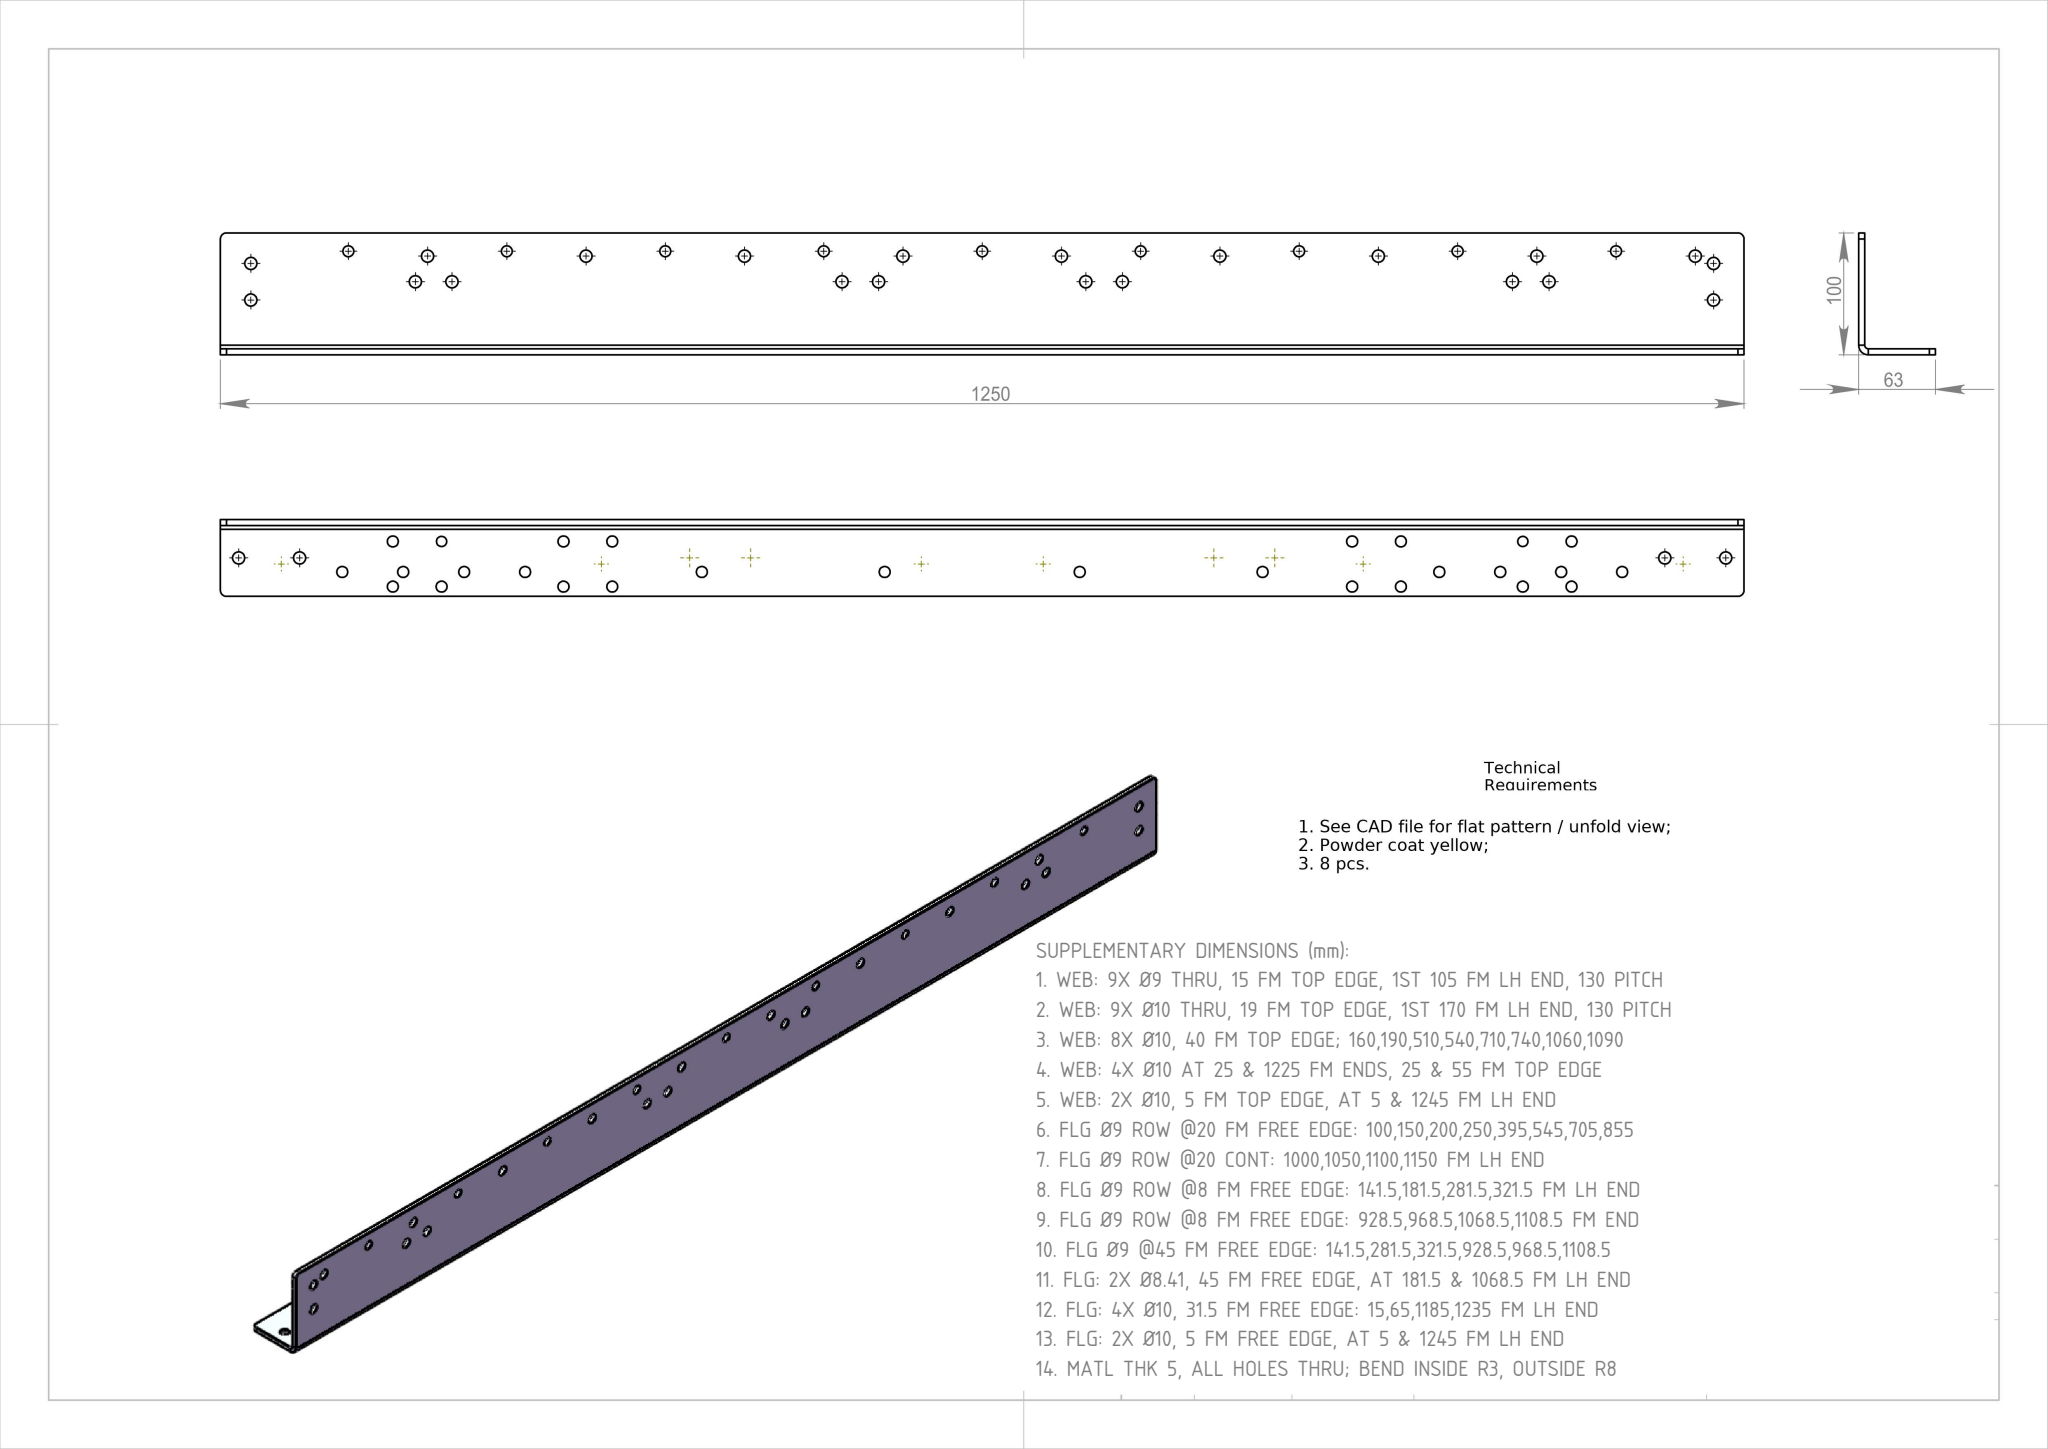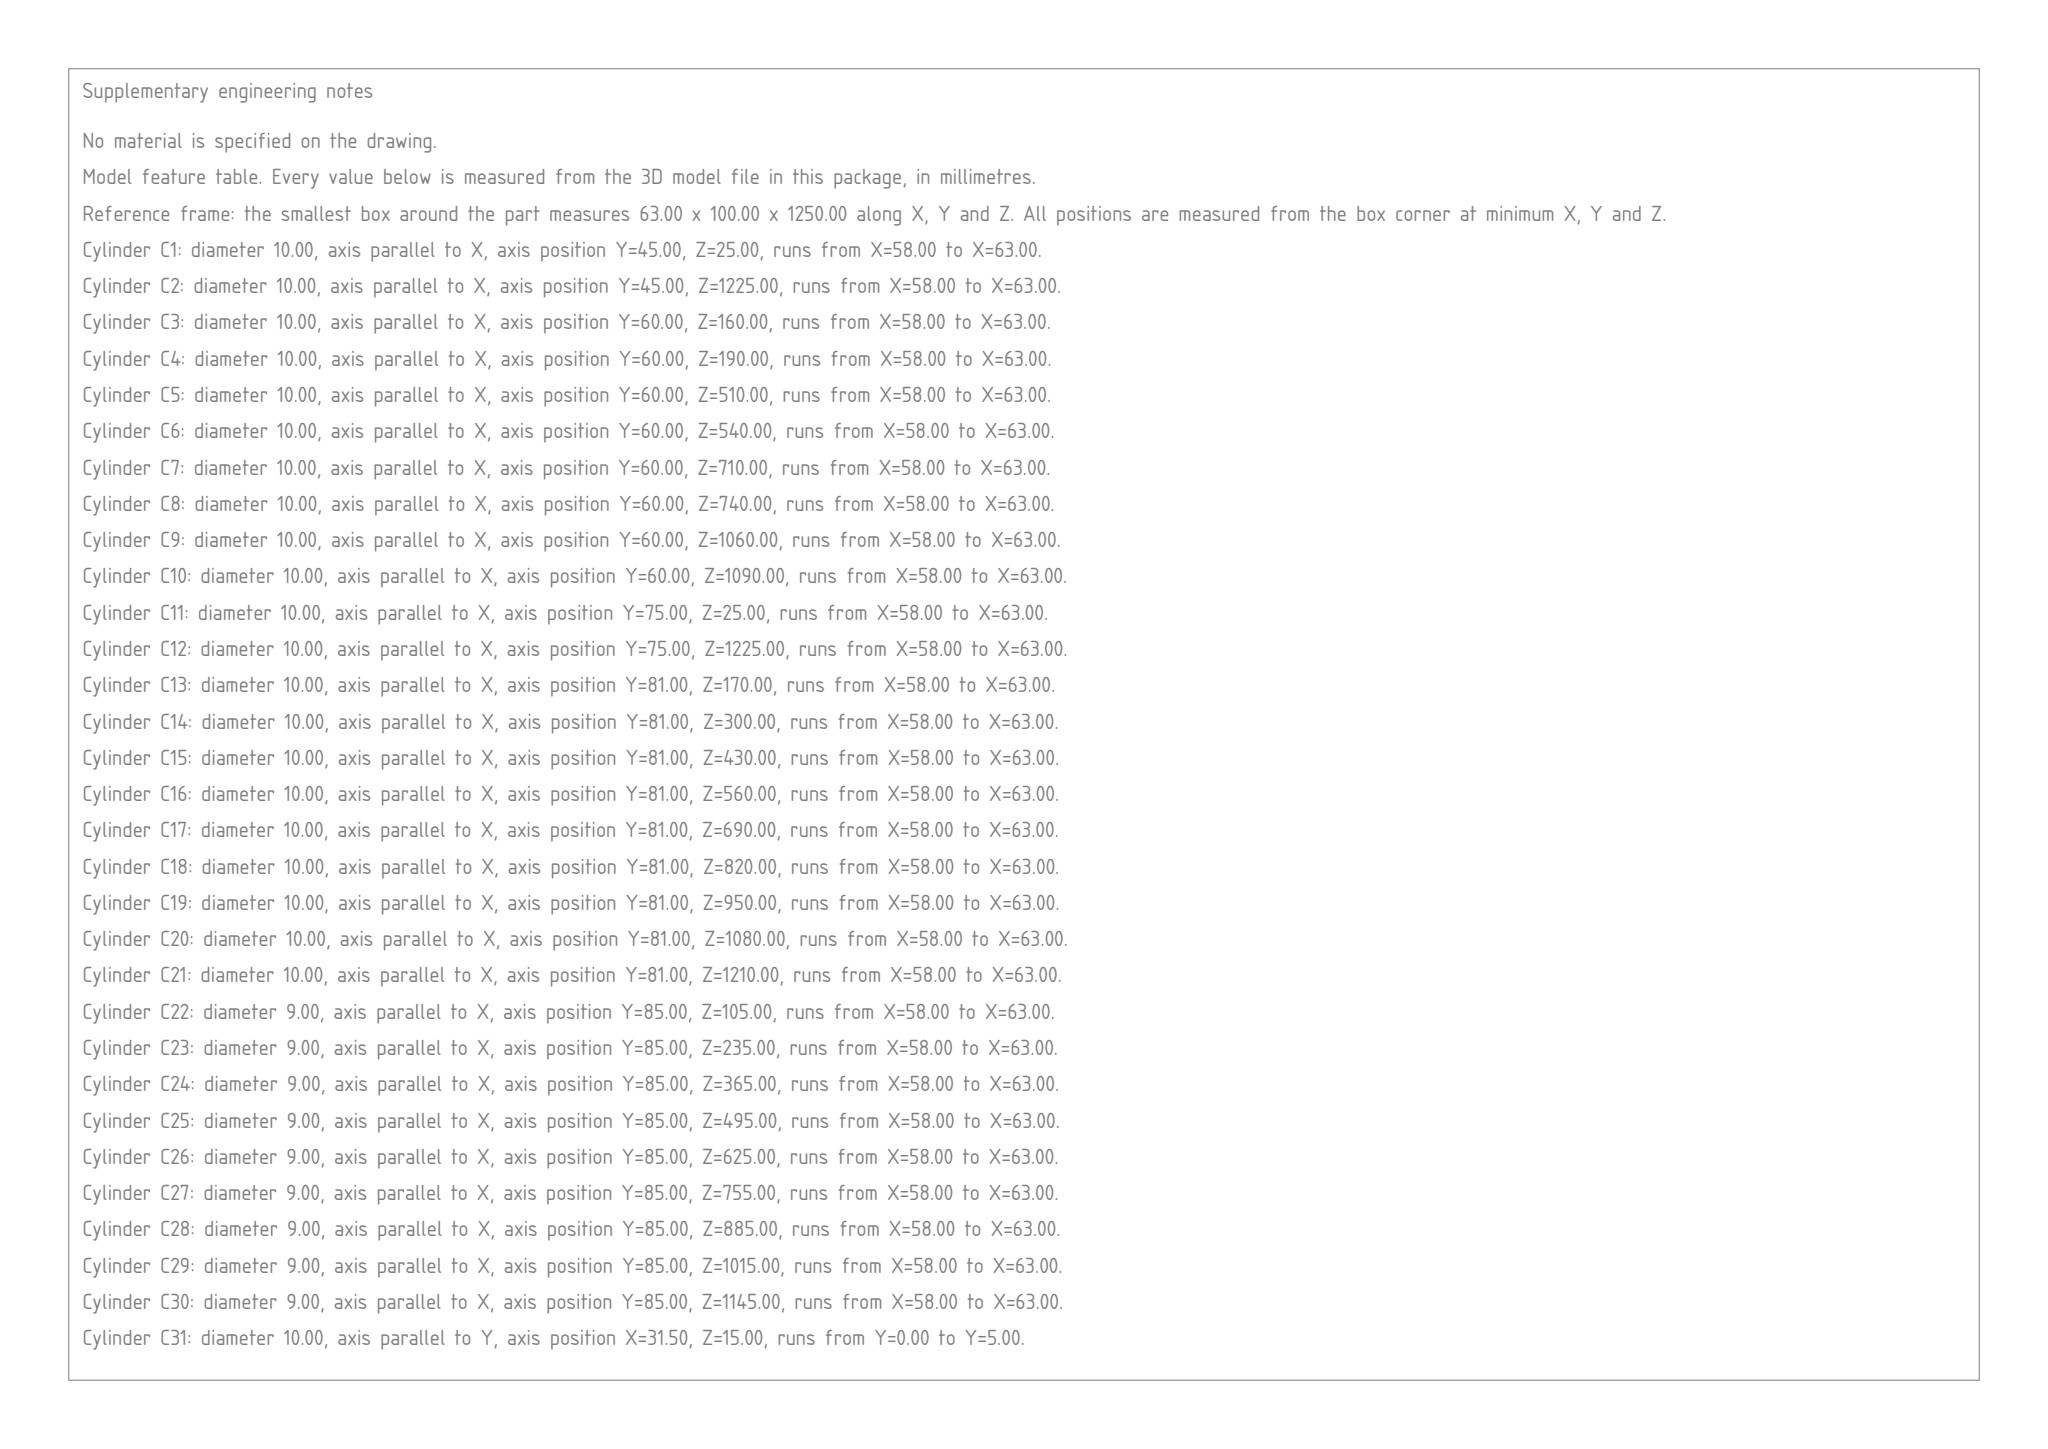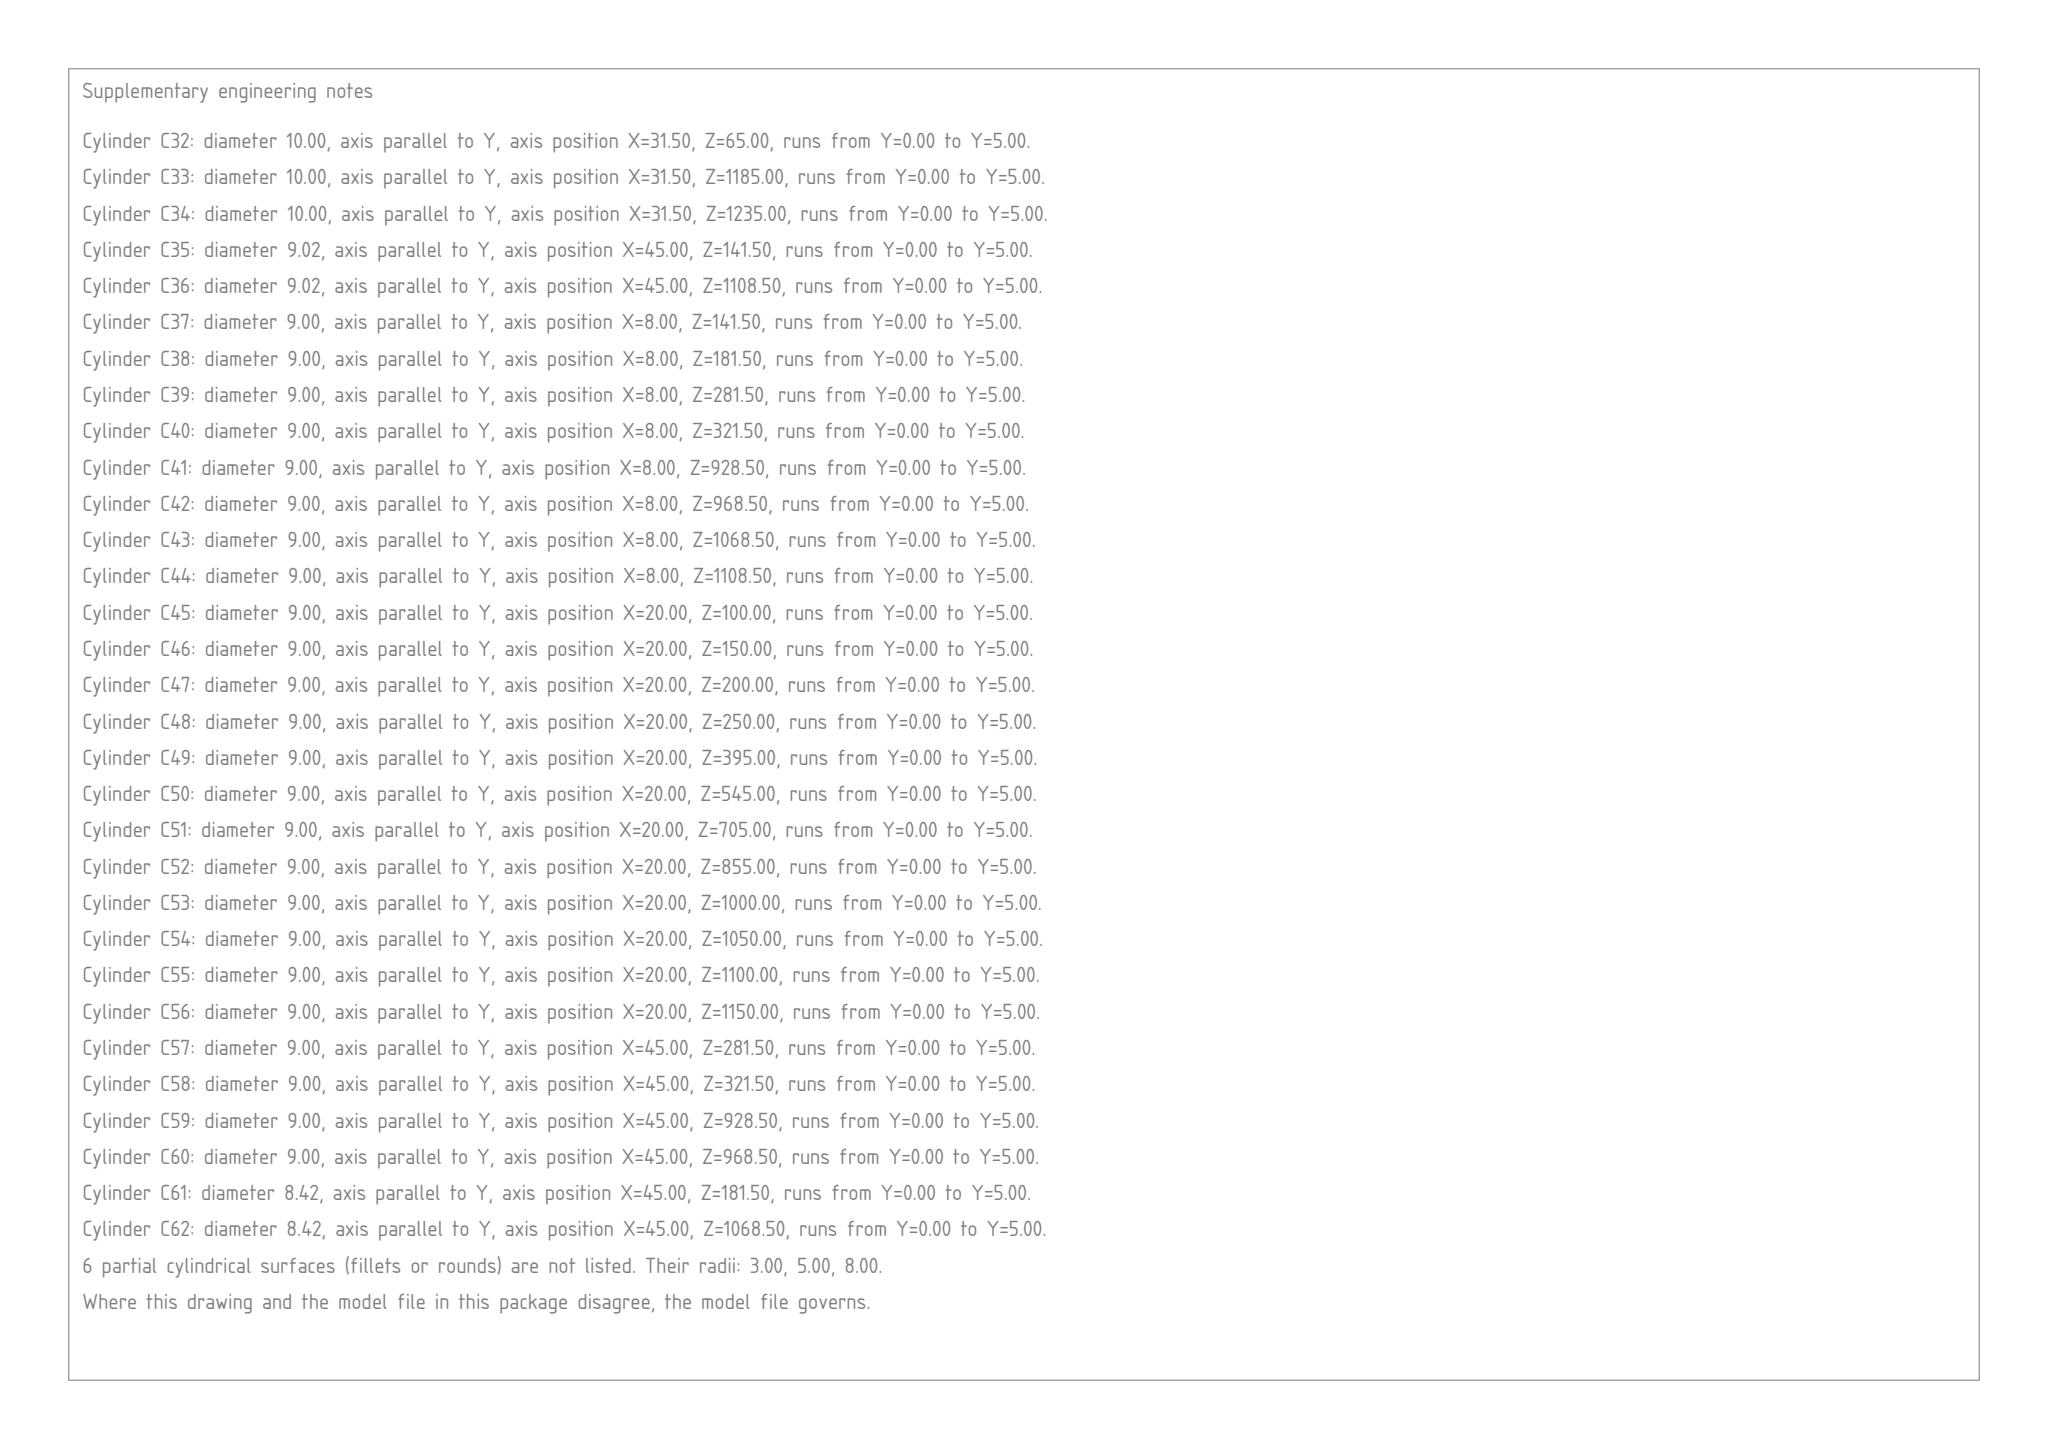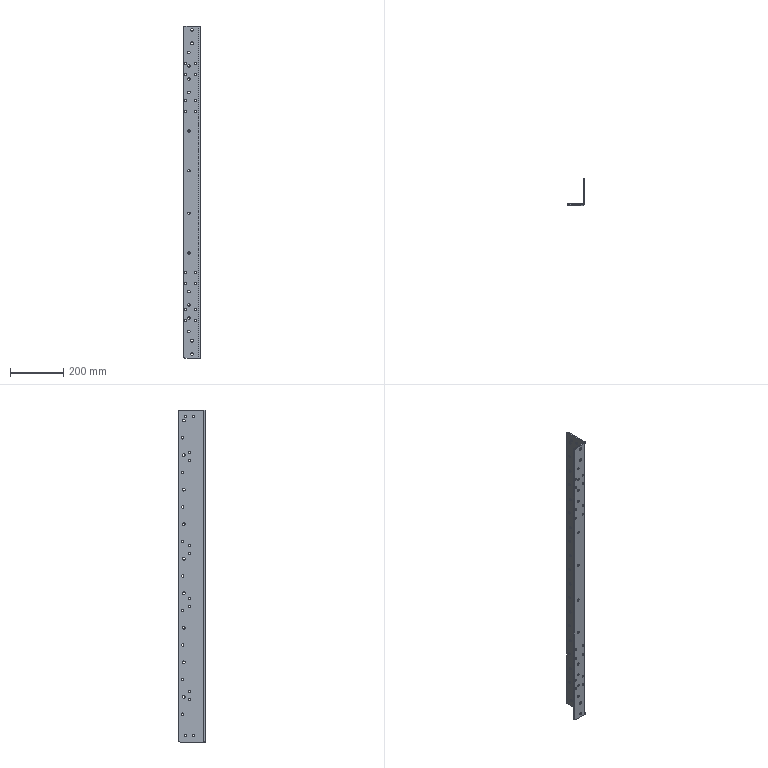Part | SolidWorks | mm | 1 solid | 142 faces | box 63 x 100 x 1250 mm | volume 951131 mm3 | cylinder 130 | plane 12 | commonest cylinder face diameters 9 x66 10 x54 8.41 x4 9.016 x4 16 x1 6 x1